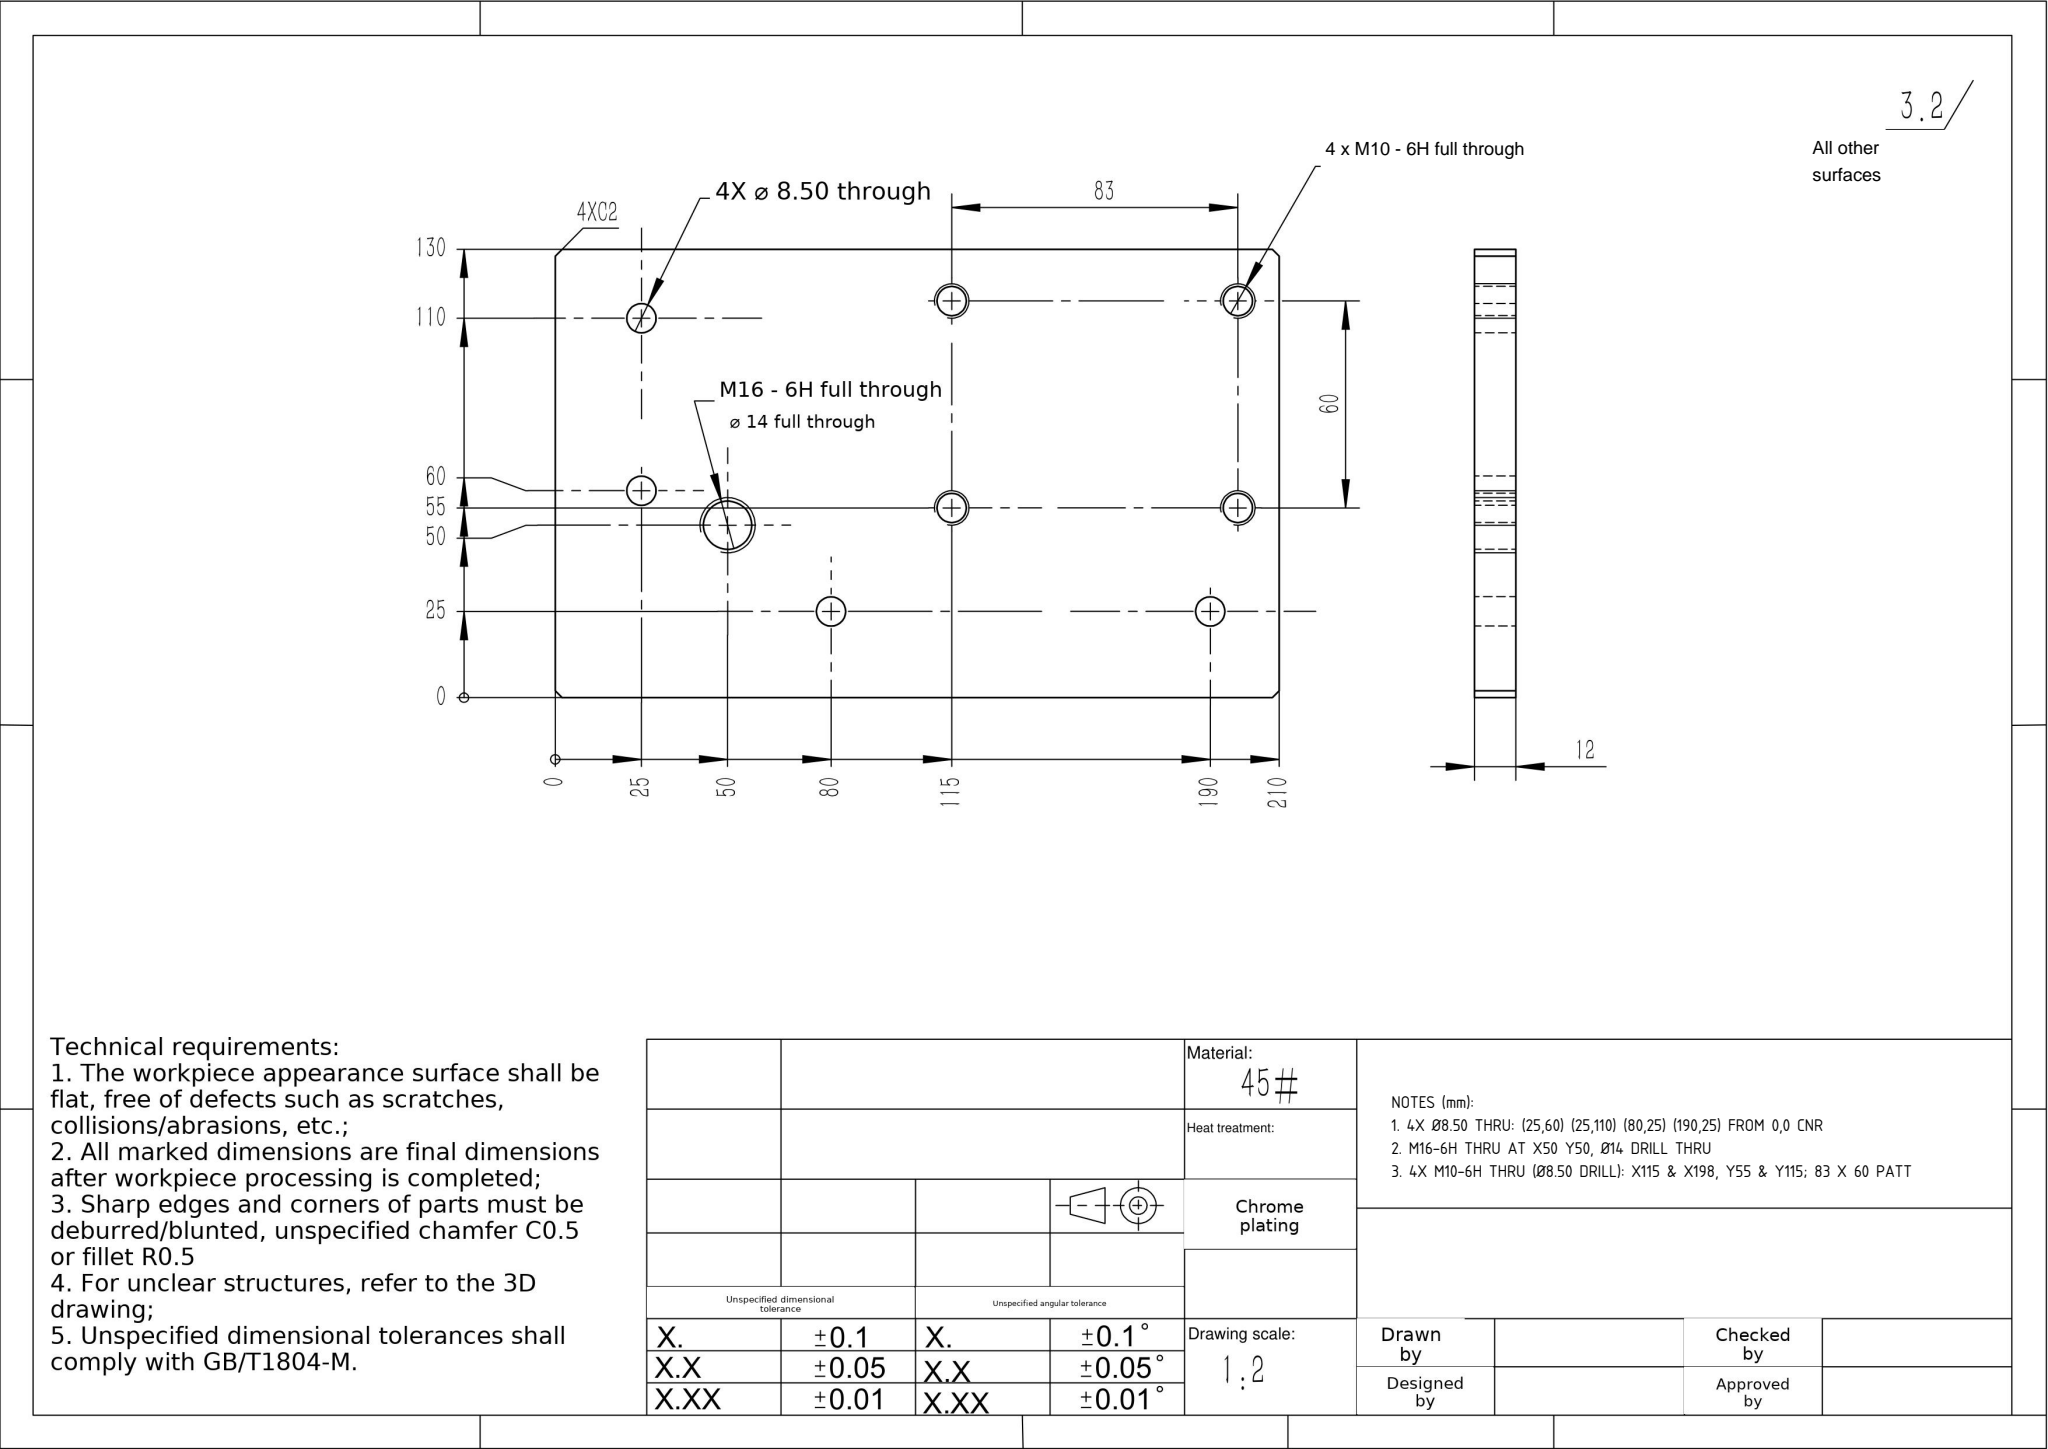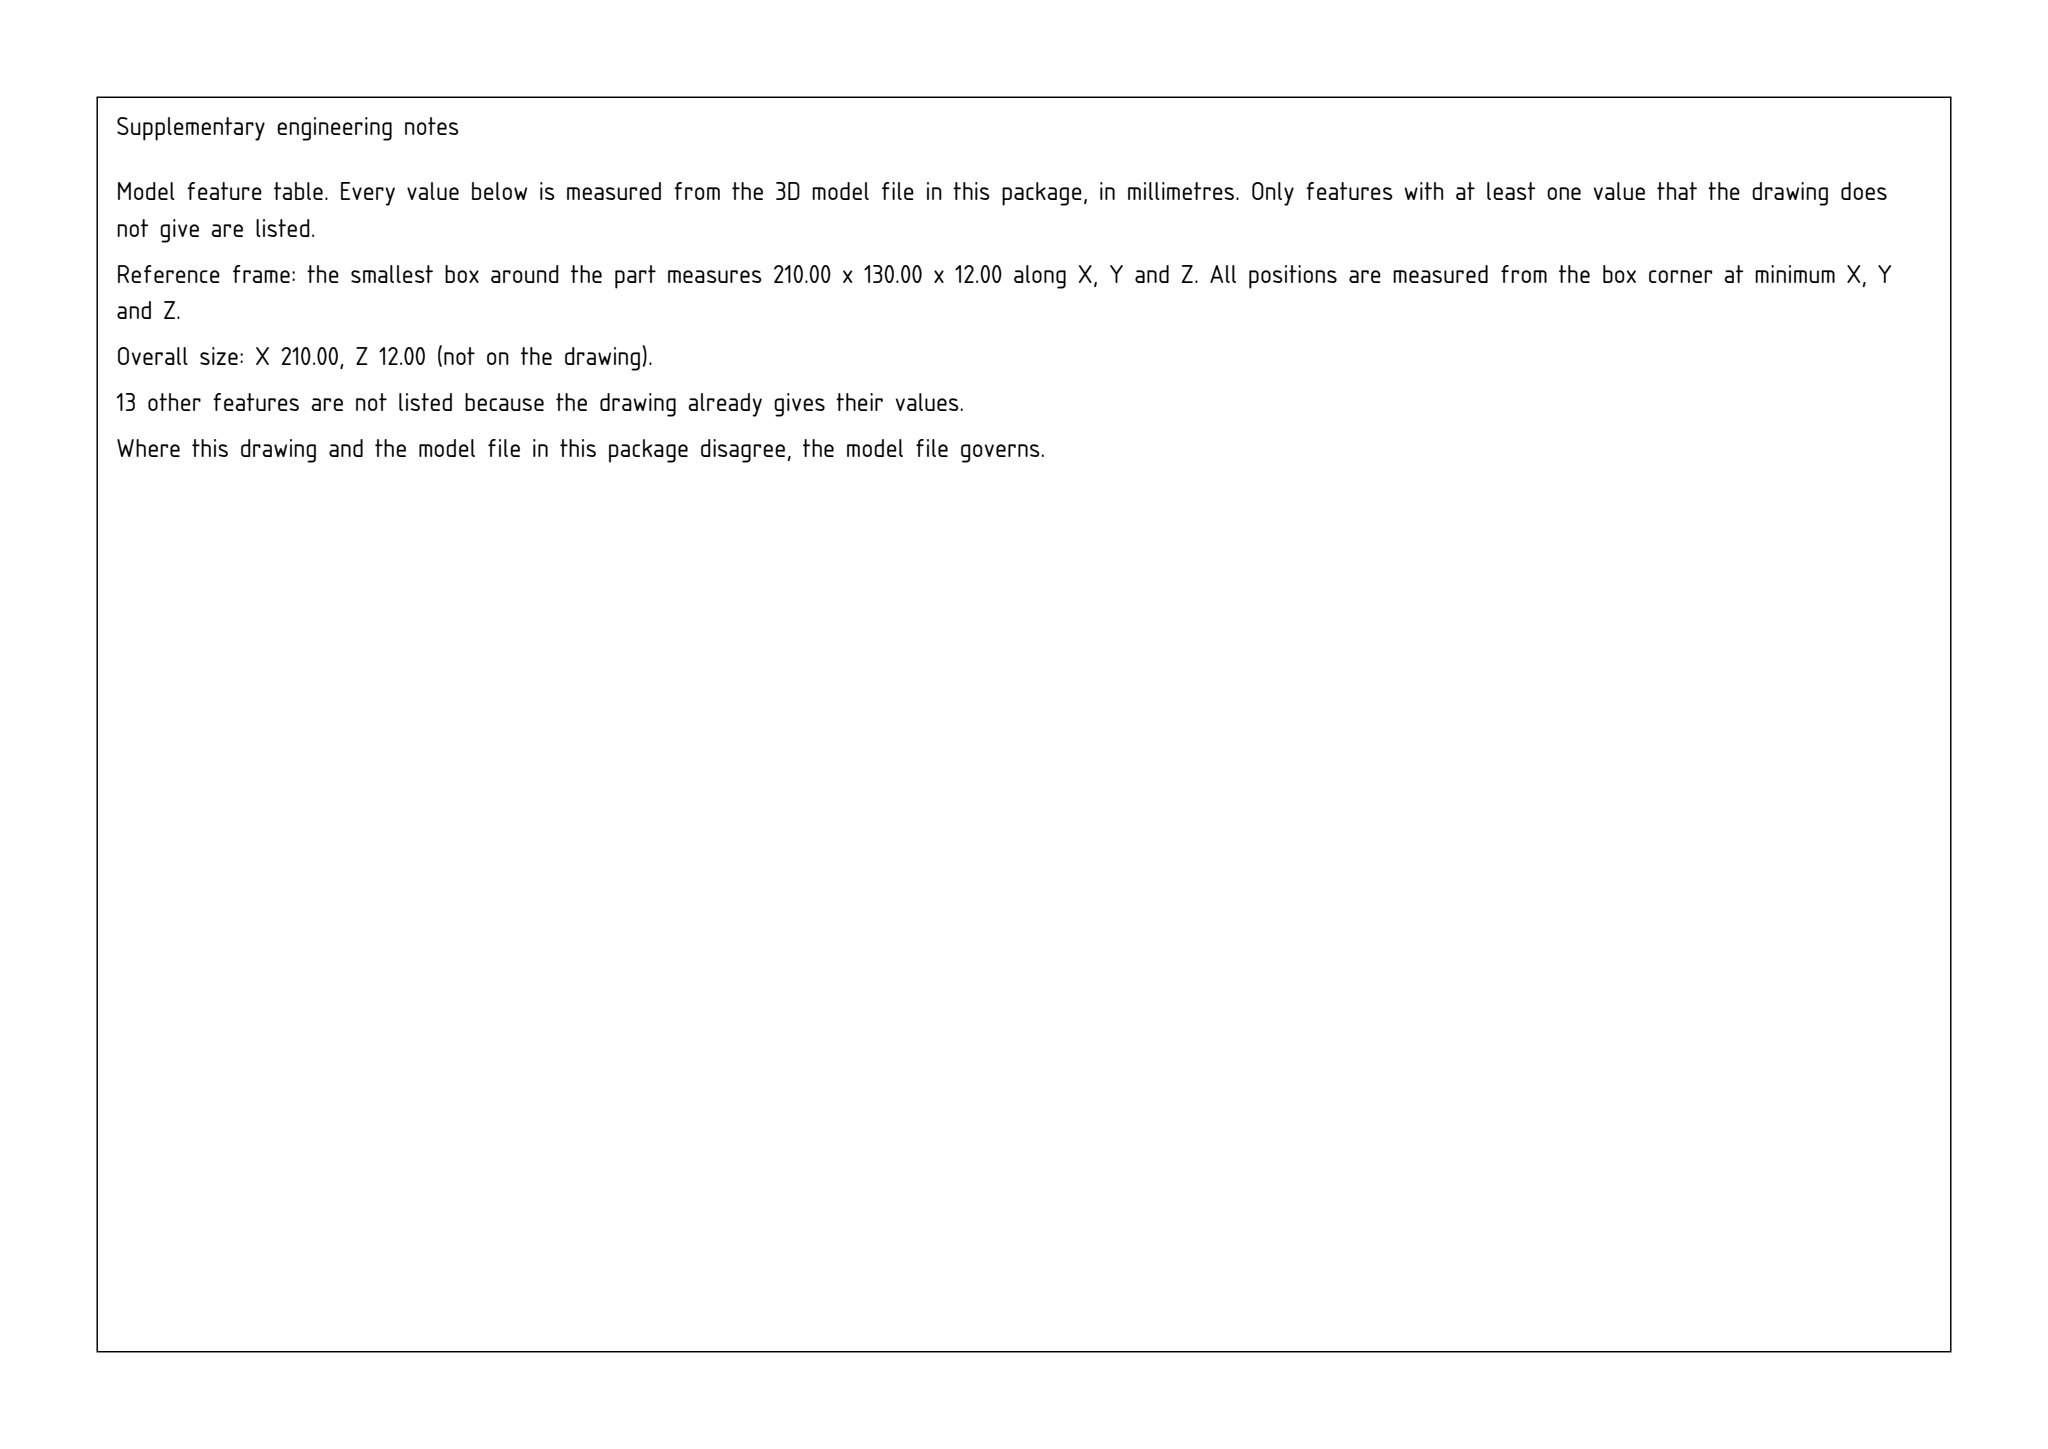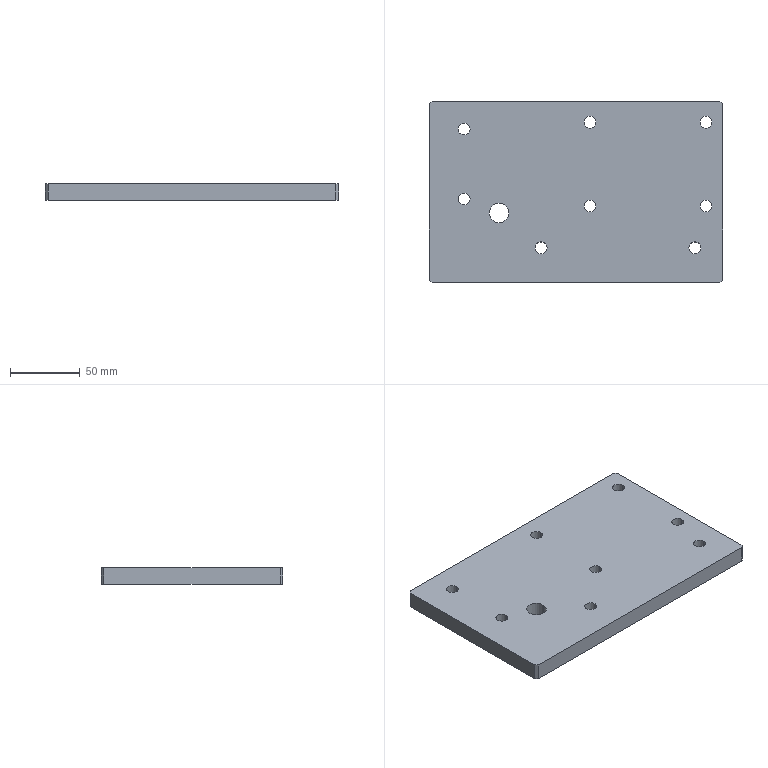Part | SolidWorks | mm | 1 solid | 28 faces | box 210 x 130 x 12 mm | volume 320209 mm3 | cylinder 18 | plane 10 | commonest cylinder face diameters 8.5 x16 14 x2
Drawing notes:
4X Ø8.50 THRU: (25,60) (25,110) (80,25) (190,25) FROM 0,0 CNR | from the solid: Ø8.5 z-axis holes at these XY, L=12 full thru, from bbox min corner
M16-6H THRU AT X50 Y50, Ø14 DRILL THRU | from the solid: Ø14 z-axis hole at [50,50], L=12 thru
4X M10-6H THRU (Ø8.50 DRILL): X115 & X198, Y55 & Y115; 83 X 60 PATT | from the solid: Ø8.5 holes at (115,55),(115,115),(198,55),(198,115); 198-115=83, 115-55=60
build123d program:
from build123d import *

# Parameters (mm, degrees)
SKETCH1_W           = 210
SKETCH1_H           = 130
BOSS_EXTRUDE1_DEPTH = 12
M16_TAPPED_HOLE1_D  = 14
CHAMFER1_SIZE       = 2
SKETCH7_R           = 4.25
CUT_EXTRUDE1_DEPTH  = 125.073
M10_TAPPED_HOLE1_D  = 8.5


with BuildPart() as part:
    # Sketch1 → Boss-Extrude1 (new body)
    with BuildSketch(Plane.XY):
        Rectangle(SKETCH1_W, SKETCH1_H)
    extrude(amount=BOSS_EXTRUDE1_DEPTH)

    # M16 Tapped Hole1 (through all)
    with Locations(Plane(origin=(-55, -15, 12), x_dir=(1, 0, 0), z_dir=(0, 0, 1))):
        with Locations((0, 0)):
            Hole(M16_TAPPED_HOLE1_D / 2)

    # Chamfer1
    chamfer1_edges = [part.edges().sort_by_distance(p)[0] for p in [
        (-105, -65, 6),
        (105, -65, 6),
        (-105, 65, 6),
        (105, 65, 6),
    ]]
    chamfer(chamfer1_edges, length=CHAMFER1_SIZE)

    # Sketch7 → Cut-Extrude1 (cut, through all)
    with BuildSketch(Plane.XY.offset(12)):
        with Locations((-80, 45)):
            Circle(SKETCH7_R)
        with Locations((-80, -5)):
            Circle(SKETCH7_R)
        with Locations((-25, -40)):
            Circle(SKETCH7_R)
        with Locations((85, -40)):
            Circle(SKETCH7_R)
    extrude(amount=-CUT_EXTRUDE1_DEPTH, mode=Mode.SUBTRACT)

    # M10 Tapped Hole1 (through all)
    with Locations(Plane(origin=(10, 50, 12), x_dir=(1, 0, 0), z_dir=(0, 0, 1))):
        with Locations((0, 0), (0, -60), (83, -60), (83, 0)):
            Hole(M10_TAPPED_HOLE1_D / 2)


solid = part.part